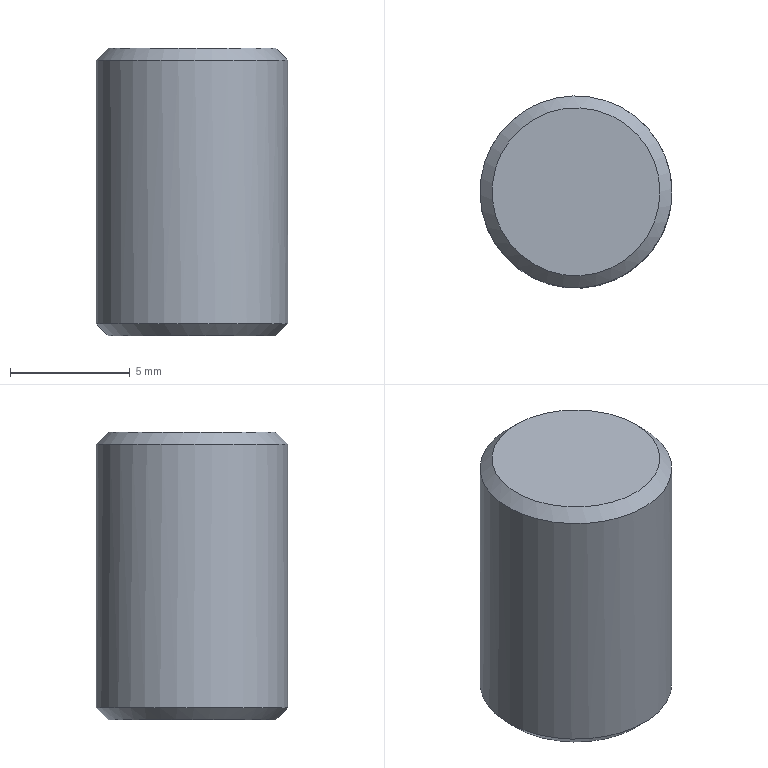Component | NX | 14_2 | 1 solid | 5 faces | box 8 x 8 x 12 mm | volume 597 mm3 | plane 2 | cone 2 | cylinder 1 | commonest cylinder face diameters 8 x1
STEP:
#1=CARTESIAN_POINT('',(0.,0.,0.));
#2=DIRECTION('',(0.,0.,1.));
#3=DIRECTION('',(1.,0.,0.));
#4=AXIS2_PLACEMENT_3D('',#1,#2,#3);
#5=CARTESIAN_POINT('',(-3.25,46.2,-36.));
#6=VERTEX_POINT('',#5);
#7=CARTESIAN_POINT('',(0.,47.5,-36.));
#8=DIRECTION('',(0.,0.,-1.));
#9=DIRECTION('',(-0.9285,-0.3714,0.));
#10=AXIS2_PLACEMENT_3D('',#7,#8,#9);
#11=CIRCLE('',#10,3.5);
#12=CARTESIAN_POINT('',(0.,47.5,-36.));
#13=DIRECTION('',(0.,0.,-1.));
#14=DIRECTION('',(-0.9285,-0.3714,0.));
#15=AXIS2_PLACEMENT_3D('',#12,#13,#14);
#16=PLANE('',#15);
#17=CARTESIAN_POINT('',(0.,0.));
#18=DIRECTION('',(1.,0.));
#19=AXIS2_PLACEMENT_2D('',#17,#18);
#20=CIRCLE('',#19,3.5);
#21=(GEOMETRIC_REPRESENTATION_CONTEXT(2)PARAMETRIC_REPRESENTATION_CONTEXT()REPRESENTATION_CONTEXT('',''));
#22=DEFINITIONAL_REPRESENTATION('',(#20),#21);
#23=PCURVE('',#16,#22);
#24=CARTESIAN_POINT('',(0.,47.5,-35.5));
#25=DIRECTION('',(0.,0.,1.));
#26=DIRECTION('',(0.9285,0.3714,0.));
#27=AXIS2_PLACEMENT_3D('',#24,#25,#26);
#28=CONICAL_SURFACE('',#27,4.,0.7854);
#29=CARTESIAN_POINT('',(9.425,-0.5));
#30=DIRECTION('',(-1.,0.));
#31=VECTOR('',#30,1.);
#32=LINE('',#29,#31);
#33=(GEOMETRIC_REPRESENTATION_CONTEXT(2)PARAMETRIC_REPRESENTATION_CONTEXT()REPRESENTATION_CONTEXT('',''));
#34=DEFINITIONAL_REPRESENTATION('',(#32),#33);
#35=PCURVE('',#28,#34);
#36=SURFACE_CURVE('',#11,(#23,#35),.PCURVE_S1.);
#37=EDGE_CURVE('',#6,#6,#36,.T.);
#38=ORIENTED_EDGE('',*,*,#37,.T.);
#39=EDGE_LOOP('',(#38));
#40=FACE_BOUND('',#39,.T.);
#41=ADVANCED_FACE('',(#40),#16,.T.);
#42=CARTESIAN_POINT('',(3.25,48.8,-24.));
#43=VERTEX_POINT('',#42);
#44=CARTESIAN_POINT('',(0.,47.5,-24.));
#45=DIRECTION('',(0.,0.,1.));
#46=DIRECTION('',(0.9285,0.3714,0.));
#47=AXIS2_PLACEMENT_3D('',#44,#45,#46);
#48=CIRCLE('',#47,3.5);
#49=CARTESIAN_POINT('',(0.,47.5,-24.));
#50=DIRECTION('',(0.,0.,1.));
#51=DIRECTION('',(0.9285,0.3714,0.));
#52=AXIS2_PLACEMENT_3D('',#49,#50,#51);
#53=PLANE('',#52);
#54=CARTESIAN_POINT('',(0.,0.));
#55=DIRECTION('',(1.,0.));
#56=AXIS2_PLACEMENT_2D('',#54,#55);
#57=CIRCLE('',#56,3.5);
#58=(GEOMETRIC_REPRESENTATION_CONTEXT(2)PARAMETRIC_REPRESENTATION_CONTEXT()REPRESENTATION_CONTEXT('',''));
#59=DEFINITIONAL_REPRESENTATION('',(#57),#58);
#60=PCURVE('',#53,#59);
#61=CARTESIAN_POINT('',(0.,47.5,-24.5));
#62=DIRECTION('',(0.,0.,-1.));
#63=DIRECTION('',(-0.9285,-0.3714,0.));
#64=AXIS2_PLACEMENT_3D('',#61,#62,#63);
#65=CONICAL_SURFACE('',#64,4.,0.7854);
#66=CARTESIAN_POINT('',(9.425,-0.5));
#67=DIRECTION('',(-1.,0.));
#68=VECTOR('',#67,1.);
#69=LINE('',#66,#68);
#70=(GEOMETRIC_REPRESENTATION_CONTEXT(2)PARAMETRIC_REPRESENTATION_CONTEXT()REPRESENTATION_CONTEXT('',''));
#71=DEFINITIONAL_REPRESENTATION('',(#69),#70);
#72=PCURVE('',#65,#71);
#73=SURFACE_CURVE('',#48,(#60,#72),.PCURVE_S1.);
#74=EDGE_CURVE('',#43,#43,#73,.T.);
#75=ORIENTED_EDGE('',*,*,#74,.T.);
#76=EDGE_LOOP('',(#75));
#77=FACE_BOUND('',#76,.T.);
#78=ADVANCED_FACE('',(#77),#53,.T.);
#79=CARTESIAN_POINT('',(3.714,48.986,-24.5));
#80=VERTEX_POINT('',#79);
#81=CARTESIAN_POINT('',(-3.714,46.014,-24.5));
#82=VERTEX_POINT('',#81);
#83=CARTESIAN_POINT('',(0.,47.5,-24.5));
#84=DIRECTION('',(0.,0.,-1.));
#85=DIRECTION('',(0.9285,0.3714,0.));
#86=AXIS2_PLACEMENT_3D('',#83,#84,#85);
#87=CIRCLE('',#86,4.);
#88=CARTESIAN_POINT('',(0.,47.5,-24.));
#89=DIRECTION('',(0.,0.,-1.));
#90=DIRECTION('',(-0.9285,-0.3714,0.));
#91=AXIS2_PLACEMENT_3D('',#88,#89,#90);
#92=CYLINDRICAL_SURFACE('',#91,4.);
#93=CARTESIAN_POINT('',(3.142,0.5));
#94=DIRECTION('',(1.,0.));
#95=VECTOR('',#94,1.);
#96=LINE('',#93,#95);
#97=(GEOMETRIC_REPRESENTATION_CONTEXT(2)PARAMETRIC_REPRESENTATION_CONTEXT()REPRESENTATION_CONTEXT('',''));
#98=DEFINITIONAL_REPRESENTATION('',(#96),#97);
#99=PCURVE('',#92,#98);
#100=CARTESIAN_POINT('',(3.142,0.));
#101=DIRECTION('',(1.,-0.));
#102=VECTOR('',#101,1.);
#103=LINE('',#100,#102);
#104=(GEOMETRIC_REPRESENTATION_CONTEXT(2)PARAMETRIC_REPRESENTATION_CONTEXT()REPRESENTATION_CONTEXT('',''));
#105=DEFINITIONAL_REPRESENTATION('',(#103),#104);
#106=PCURVE('',#65,#105);
#107=SURFACE_CURVE('',#87,(#99,#106),.PCURVE_S1.);
#108=EDGE_CURVE('',#80,#82,#107,.T.);
#109=ORIENTED_EDGE('',*,*,#108,.T.);
#110=CARTESIAN_POINT('',(-3.714,46.014,-35.5));
#111=VERTEX_POINT('',#110);
#112=CARTESIAN_POINT('',(-3.714,46.014,-24.5));
#113=CARTESIAN_POINT('',(-3.714,46.014,-35.5));
#114=B_SPLINE_CURVE_WITH_KNOTS('',1,(#112,#113),.UNSPECIFIED.,.F.,.F.,(2,2),(0.5,11.5),.PIECEWISE_BEZIER_KNOTS.);
#115=CARTESIAN_POINT('',(6.283,0.));
#116=DIRECTION('',(0.,1.));
#117=VECTOR('',#116,1.);
#118=LINE('',#115,#117);
#119=(GEOMETRIC_REPRESENTATION_CONTEXT(2)PARAMETRIC_REPRESENTATION_CONTEXT()REPRESENTATION_CONTEXT('',''));
#120=DEFINITIONAL_REPRESENTATION('',(#118),#119);
#121=PCURVE('',#92,#120);
#122=CARTESIAN_POINT('',(0.,0.));
#123=DIRECTION('',(0.,1.));
#124=VECTOR('',#123,1.);
#125=LINE('',#122,#124);
#126=(GEOMETRIC_REPRESENTATION_CONTEXT(2)PARAMETRIC_REPRESENTATION_CONTEXT()REPRESENTATION_CONTEXT('',''));
#127=DEFINITIONAL_REPRESENTATION('',(#125),#126);
#128=PCURVE('',#92,#127);
#129=SEAM_CURVE('',#114,(#121,#128),.PCURVE_S1.);
#130=EDGE_CURVE('',#82,#111,#129,.T.);
#131=ORIENTED_EDGE('',*,*,#130,.T.);
#132=CARTESIAN_POINT('',(0.,47.5,-35.5));
#133=DIRECTION('',(0.,0.,1.));
#134=DIRECTION('',(-0.9285,-0.3714,0.));
#135=AXIS2_PLACEMENT_3D('',#132,#133,#134);
#136=CIRCLE('',#135,4.);
#137=CARTESIAN_POINT('',(6.283,11.5));
#138=DIRECTION('',(-1.,0.));
#139=VECTOR('',#138,1.);
#140=LINE('',#137,#139);
#141=(GEOMETRIC_REPRESENTATION_CONTEXT(2)PARAMETRIC_REPRESENTATION_CONTEXT()REPRESENTATION_CONTEXT('',''));
#142=DEFINITIONAL_REPRESENTATION('',(#140),#141);
#143=PCURVE('',#92,#142);
#144=CARTESIAN_POINT('',(3.142,-0.));
#145=DIRECTION('',(1.,0.));
#146=VECTOR('',#145,1.);
#147=LINE('',#144,#146);
#148=(GEOMETRIC_REPRESENTATION_CONTEXT(2)PARAMETRIC_REPRESENTATION_CONTEXT()REPRESENTATION_CONTEXT('',''));
#149=DEFINITIONAL_REPRESENTATION('',(#147),#148);
#150=PCURVE('',#28,#149);
#151=SURFACE_CURVE('',#136,(#143,#150),.PCURVE_S1.);
#152=EDGE_CURVE('',#111,#111,#151,.T.);
#153=ORIENTED_EDGE('',*,*,#152,.T.);
#154=ORIENTED_EDGE('',*,*,#130,.F.);
#155=CARTESIAN_POINT('',(0.,47.5,-24.5));
#156=DIRECTION('',(0.,0.,-1.));
#157=DIRECTION('',(0.9285,0.3714,0.));
#158=AXIS2_PLACEMENT_3D('',#155,#156,#157);
#159=CIRCLE('',#158,4.);
#160=CARTESIAN_POINT('',(-3.142,0.5));
#161=DIRECTION('',(1.,0.));
#162=VECTOR('',#161,1.);
#163=LINE('',#160,#162);
#164=(GEOMETRIC_REPRESENTATION_CONTEXT(2)PARAMETRIC_REPRESENTATION_CONTEXT()REPRESENTATION_CONTEXT('',''));
#165=DEFINITIONAL_REPRESENTATION('',(#163),#164);
#166=PCURVE('',#92,#165);
#167=CARTESIAN_POINT('',(3.142,-0.));
#168=DIRECTION('',(1.,0.));
#169=VECTOR('',#168,1.);
#170=LINE('',#167,#169);
#171=(GEOMETRIC_REPRESENTATION_CONTEXT(2)PARAMETRIC_REPRESENTATION_CONTEXT()REPRESENTATION_CONTEXT('',''));
#172=DEFINITIONAL_REPRESENTATION('',(#170),#171);
#173=PCURVE('',#65,#172);
#174=SURFACE_CURVE('',#159,(#166,#173),.PCURVE_S1.);
#175=EDGE_CURVE('',#82,#80,#174,.T.);
#176=ORIENTED_EDGE('',*,*,#175,.T.);
#177=EDGE_LOOP('',(#109,#131,#153,#154,#176));
#178=FACE_BOUND('',#177,.T.);
#179=ADVANCED_FACE('',(#178),#92,.T.);
#180=ORIENTED_EDGE('',*,*,#74,.F.);
#181=CARTESIAN_POINT('',(3.25,48.8,-24.));
#182=CARTESIAN_POINT('',(3.714,48.986,-24.5));
#183=B_SPLINE_CURVE_WITH_KNOTS('',1,(#181,#182),.UNSPECIFIED.,.F.,.F.,(2,2),(-0.7071,0.),.PIECEWISE_BEZIER_KNOTS.);
#184=CARTESIAN_POINT('',(9.425,0.));
#185=DIRECTION('',(0.,1.));
#186=VECTOR('',#185,1.);
#187=LINE('',#184,#186);
#188=(GEOMETRIC_REPRESENTATION_CONTEXT(2)PARAMETRIC_REPRESENTATION_CONTEXT()REPRESENTATION_CONTEXT('',''));
#189=DEFINITIONAL_REPRESENTATION('',(#187),#188);
#190=PCURVE('',#65,#189);
#191=CARTESIAN_POINT('',(3.142,0.));
#192=DIRECTION('',(0.,1.));
#193=VECTOR('',#192,1.);
#194=LINE('',#191,#193);
#195=(GEOMETRIC_REPRESENTATION_CONTEXT(2)PARAMETRIC_REPRESENTATION_CONTEXT()REPRESENTATION_CONTEXT('',''));
#196=DEFINITIONAL_REPRESENTATION('',(#194),#195);
#197=PCURVE('',#65,#196);
#198=SEAM_CURVE('',#183,(#190,#197),.PCURVE_S1.);
#199=EDGE_CURVE('',#43,#80,#198,.T.);
#200=ORIENTED_EDGE('',*,*,#199,.T.);
#201=ORIENTED_EDGE('',*,*,#175,.F.);
#202=ORIENTED_EDGE('',*,*,#108,.F.);
#203=ORIENTED_EDGE('',*,*,#199,.F.);
#204=EDGE_LOOP('',(#180,#200,#201,#202,#203));
#205=FACE_BOUND('',#204,.T.);
#206=ADVANCED_FACE('',(#205),#65,.T.);
#207=ORIENTED_EDGE('',*,*,#37,.F.);
#208=CARTESIAN_POINT('',(-3.25,46.2,-36.));
#209=CARTESIAN_POINT('',(-3.714,46.014,-35.5));
#210=B_SPLINE_CURVE_WITH_KNOTS('',1,(#208,#209),.UNSPECIFIED.,.F.,.F.,(2,2),(-0.7071,-0.),.PIECEWISE_BEZIER_KNOTS.);
#211=CARTESIAN_POINT('',(9.425,0.));
#212=DIRECTION('',(0.,1.));
#213=VECTOR('',#212,1.);
#214=LINE('',#211,#213);
#215=(GEOMETRIC_REPRESENTATION_CONTEXT(2)PARAMETRIC_REPRESENTATION_CONTEXT()REPRESENTATION_CONTEXT('',''));
#216=DEFINITIONAL_REPRESENTATION('',(#214),#215);
#217=PCURVE('',#28,#216);
#218=CARTESIAN_POINT('',(3.142,0.));
#219=DIRECTION('',(0.,1.));
#220=VECTOR('',#219,1.);
#221=LINE('',#218,#220);
#222=(GEOMETRIC_REPRESENTATION_CONTEXT(2)PARAMETRIC_REPRESENTATION_CONTEXT()REPRESENTATION_CONTEXT('',''));
#223=DEFINITIONAL_REPRESENTATION('',(#221),#222);
#224=PCURVE('',#28,#223);
#225=SEAM_CURVE('',#210,(#217,#224),.PCURVE_S1.);
#226=EDGE_CURVE('',#6,#111,#225,.T.);
#227=ORIENTED_EDGE('',*,*,#226,.T.);
#228=ORIENTED_EDGE('',*,*,#152,.F.);
#229=ORIENTED_EDGE('',*,*,#226,.F.);
#230=EDGE_LOOP('',(#207,#227,#228,#229));
#231=FACE_BOUND('',#230,.T.);
#232=ADVANCED_FACE('',(#231),#28,.T.);
#233=CLOSED_SHELL('',(#41,#78,#179,#206,#232));
#234=MANIFOLD_SOLID_BREP('',#233);
#235=(LENGTH_UNIT()NAMED_UNIT(*)SI_UNIT(.MILLI.,.METRE.));
#236=UNCERTAINTY_MEASURE_WITH_UNIT(LENGTH_MEASURE(0.00001),#235,'','');
#237=(NAMED_UNIT(*)PLANE_ANGLE_UNIT()SI_UNIT($,.RADIAN.));
#238=(NAMED_UNIT(*)SI_UNIT($,.STERADIAN.)SOLID_ANGLE_UNIT());
#239=(GEOMETRIC_REPRESENTATION_CONTEXT(3)GLOBAL_UNCERTAINTY_ASSIGNED_CONTEXT((#236))GLOBAL_UNIT_ASSIGNED_CONTEXT((#235,#237,#238))REPRESENTATION_CONTEXT('',''));
#240=ADVANCED_BREP_SHAPE_REPRESENTATION('',(#4,#234),#239);